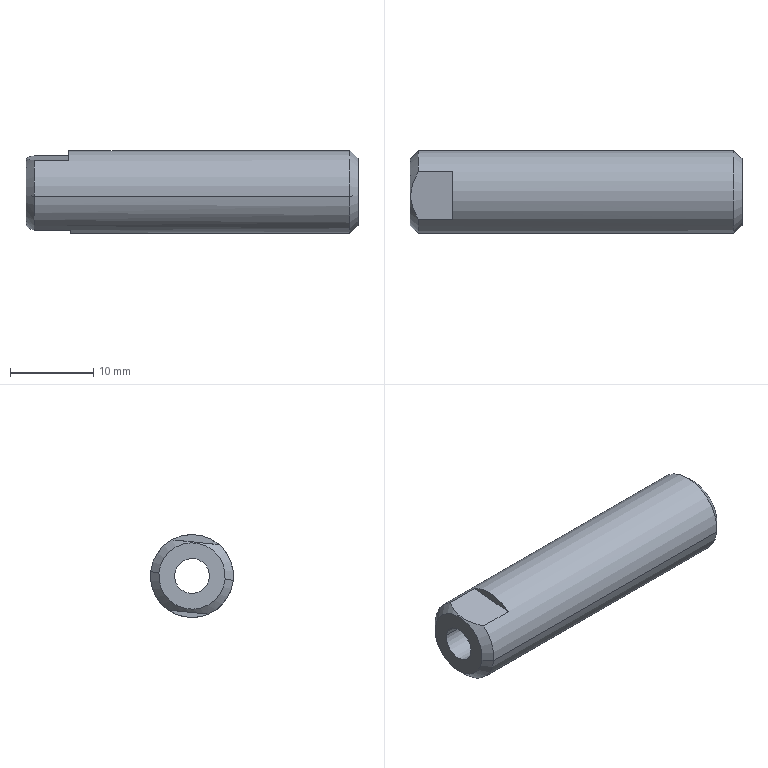Component | SolidWorks | CHEN123-AA-29-1 | 1 solid | 14 faces | box 40 x 10 x 10 mm | volume 2533 mm3 | plane 6 | cylinder 4 | cone 4 | commonest cylinder face diameters 4.2 x2 10 x2
build123d program:
from build123d import *

# Parameters (mm, degrees)
SKETCH1_R               = 5
BOSS_EXTRUDE1_DEPTH     = 40
CHAMFER1_SIZE           = 1
CUT_EXTRUDE1_DEPTH      = 41.62
CUT_EXTRUDE1_DEPTH_BACK = 41.62
SKETCH2_W               = 12.006
SKETCH2_H               = 4.106
SKETCH2_W_2             = 11.65
SKETCH2_H_2             = 2.222
M5_TAPPED_HOLE1_D       = 4.2


with BuildPart() as part:
    # Sketch1 → Boss-Extrude1 (new body)
    with BuildSketch(Plane.XY):
        Circle(SKETCH1_R)
    extrude(amount=BOSS_EXTRUDE1_DEPTH)

    # Chamfer1
    chamfer1_edges = [part.edges().sort_by_distance(p)[0] for p in [
        (-5, 0, 0),
        (-5, 0, 40),
    ]]
    chamfer(chamfer1_edges, length=CHAMFER1_SIZE)

    # Sketch2 → Cut-Extrude1 (cut, two sides: drawn at the far end of the back side and taken through both)
    with BuildSketch(Plane(origin=(0, 0, 0), x_dir=(0, 0, -1), z_dir=(1, 0, 0)).offset(-CUT_EXTRUDE1_DEPTH_BACK)):
        with Locations((-40.625, 6.426)):
            Rectangle(SKETCH2_W, SKETCH2_H)
        with Locations((-40.659, -5.201)):
            Rectangle(SKETCH2_W_2, SKETCH2_H_2)
    extrude(amount=CUT_EXTRUDE1_DEPTH + CUT_EXTRUDE1_DEPTH_BACK, mode=Mode.SUBTRACT)

    # M5 Tapped Hole1 (through all)
    with Locations(Plane.XY.offset(40)):
        with Locations((0, 0)):
            Hole(M5_TAPPED_HOLE1_D / 2)


solid = part.part

# Placed as in the assembly
solid = solid.moved(Location((20, -45.999, -230), (-167.254, -90, -83.091)))
STEP:
#1=COLOUR_RGB('',0.7922,0.8196,0.9333);
#2=FILL_AREA_STYLE_COLOUR('',#1);
#3=FILL_AREA_STYLE('',(#2));
#4=SURFACE_STYLE_FILL_AREA(#3);
#5=SURFACE_SIDE_STYLE('',(#4));
#6=SURFACE_STYLE_USAGE(.BOTH.,#5);
#7=PRESENTATION_STYLE_ASSIGNMENT((#6));
#8=CARTESIAN_POINT('',(0.7874,-1.893,-9.064));
#9=VERTEX_POINT('',#8);
#10=CARTESIAN_POINT('',(0.7874,-1.729,-9.047));
#11=VERTEX_POINT('',#10);
#12=CARTESIAN_POINT('',(0.7874,-1.811,-9.055));
#13=DIRECTION('',(-1.,0.,0.));
#14=DIRECTION('',(0.,0.9948,0.1017));
#15=AXIS2_PLACEMENT_3D('',#12,#13,#14);
#16=CIRCLE('',#15,0.08268);
#17=EDGE_CURVE('',#9,#11,#16,.T.);
#18=ORIENTED_EDGE('',*,*,#17,.F.);
#19=CARTESIAN_POINT('',(-0.7874,-1.893,-9.064));
#20=VERTEX_POINT('',#19);
#21=CARTESIAN_POINT('',(-0.7874,-1.893,-9.064));
#22=DIRECTION('',(-1.,0.,0.));
#23=VECTOR('',#22,39.37);
#24=LINE('',#21,#23);
#25=EDGE_CURVE('',#9,#20,#24,.T.);
#26=ORIENTED_EDGE('',*,*,#25,.T.);
#27=CARTESIAN_POINT('',(-0.7874,-1.729,-9.047));
#28=VERTEX_POINT('',#27);
#29=CARTESIAN_POINT('',(-0.7874,-1.811,-9.055));
#30=DIRECTION('',(-1.,0.,0.));
#31=DIRECTION('',(0.,0.9948,0.1017));
#32=AXIS2_PLACEMENT_3D('',#29,#30,#31);
#33=CIRCLE('',#32,0.08268);
#34=EDGE_CURVE('',#20,#28,#33,.T.);
#35=ORIENTED_EDGE('',*,*,#34,.T.);
#36=CARTESIAN_POINT('',(-0.7874,-1.729,-9.047));
#37=DIRECTION('',(-1.,0.,0.));
#38=VECTOR('',#37,39.37);
#39=LINE('',#36,#38);
#40=EDGE_CURVE('',#11,#28,#39,.T.);
#41=ORIENTED_EDGE('',*,*,#40,.F.);
#42=EDGE_LOOP('',(#18,#26,#35,#41));
#43=FACE_OUTER_BOUND('',#42,.T.);
#44=CARTESIAN_POINT('',(-0.7874,-1.811,-9.055));
#45=DIRECTION('',(-1.,0.,0.));
#46=DIRECTION('',(0.,0.9948,0.1017));
#47=AXIS2_PLACEMENT_3D('',#44,#45,#46);
#48=CYLINDRICAL_SURFACE('',#47,0.08268);
#49=ADVANCED_FACE('',(#43),#48,.F.);
#50=CARTESIAN_POINT('',(-0.7874,-1.654,-9.039));
#51=VERTEX_POINT('',#50);
#52=CARTESIAN_POINT('',(-0.7874,-1.968,-9.071));
#53=VERTEX_POINT('',#52);
#54=CARTESIAN_POINT('',(-0.7874,-1.811,-9.055));
#55=DIRECTION('',(-1.,0.,0.));
#56=DIRECTION('',(0.,0.9948,0.1017));
#57=AXIS2_PLACEMENT_3D('',#54,#55,#56);
#58=CIRCLE('',#57,0.1575);
#59=EDGE_CURVE('',#51,#53,#58,.T.);
#60=ORIENTED_EDGE('',*,*,#59,.F.);
#61=CARTESIAN_POINT('',(-0.7481,-1.615,-9.035));
#62=VERTEX_POINT('',#61);
#63=CARTESIAN_POINT('',(-0.7874,-1.654,-9.039));
#64=DIRECTION('',(0.7071,0.7034,0.07191));
#65=VECTOR('',#64,39.37);
#66=LINE('',#63,#65);
#67=EDGE_CURVE('',#51,#62,#66,.T.);
#68=ORIENTED_EDGE('',*,*,#67,.T.);
#69=CARTESIAN_POINT('',(-0.7481,-1.699,-9.217));
#70=VERTEX_POINT('',#69);
#71=CARTESIAN_POINT('',(-0.7481,-1.811,-9.055));
#72=DIRECTION('',(1.,0.,0.));
#73=DIRECTION('',(0.,0.9948,0.1017));
#74=AXIS2_PLACEMENT_3D('',#71,#72,#73);
#75=CIRCLE('',#74,0.1969);
#76=EDGE_CURVE('',#70,#62,#75,.T.);
#77=ORIENTED_EDGE('',*,*,#76,.F.);
#78=CARTESIAN_POINT('',(-0.7481,-1.888,-9.236));
#79=VERTEX_POINT('',#78);
#80=CARTESIAN_POINT('',(-0.7481,-1.888,-9.236));
#81=CARTESIAN_POINT('',(-0.7552,-1.874,-9.235));
#82=CARTESIAN_POINT('',(-0.7615,-1.858,-9.233));
#83=CARTESIAN_POINT('',(-0.7702,-1.826,-9.23));
#84=CARTESIAN_POINT('',(-0.7727,-1.81,-9.228));
#85=CARTESIAN_POINT('',(-0.7727,-1.777,-9.225));
#86=CARTESIAN_POINT('',(-0.7702,-1.761,-9.223));
#87=CARTESIAN_POINT('',(-0.7637,-1.737,-9.221));
#88=CARTESIAN_POINT('',(-0.761,-1.729,-9.22));
#89=CARTESIAN_POINT('',(-0.755,-1.713,-9.218));
#90=CARTESIAN_POINT('',(-0.7516,-1.706,-9.217));
#91=CARTESIAN_POINT('',(-0.7481,-1.699,-9.217));
#92=B_SPLINE_CURVE_WITH_KNOTS('',3,(#80,#81,#82,#83,#84,#85,#86,#87,#88,#89,#90,#91),.UNSPECIFIED.,.F.,.F.,(4,2,2,2,2,4),(0.003135,0.004387,0.005639,0.006891,0.007517,0.008143),.UNSPECIFIED.);
#93=EDGE_CURVE('',#79,#70,#92,.T.);
#94=ORIENTED_EDGE('',*,*,#93,.F.);
#95=CARTESIAN_POINT('',(-0.7481,-2.007,-9.075));
#96=VERTEX_POINT('',#95);
#97=CARTESIAN_POINT('',(-0.7481,-1.811,-9.055));
#98=DIRECTION('',(1.,0.,0.));
#99=DIRECTION('',(0.,0.9948,0.1017));
#100=AXIS2_PLACEMENT_3D('',#97,#98,#99);
#101=CIRCLE('',#100,0.1969);
#102=EDGE_CURVE('',#96,#79,#101,.T.);
#103=ORIENTED_EDGE('',*,*,#102,.F.);
#104=CARTESIAN_POINT('',(-0.7874,-1.968,-9.071));
#105=DIRECTION('',(0.7071,-0.7034,-0.07191));
#106=VECTOR('',#105,39.37);
#107=LINE('',#104,#106);
#108=EDGE_CURVE('',#53,#96,#107,.T.);
#109=ORIENTED_EDGE('',*,*,#108,.F.);
#110=EDGE_LOOP('',(#60,#68,#77,#94,#103,#109));
#111=FACE_OUTER_BOUND('',#110,.T.);
#112=CARTESIAN_POINT('',(-0.7874,-1.811,-9.055));
#113=DIRECTION('',(1.,0.,0.));
#114=DIRECTION('',(0.,-0.9948,-0.1017));
#115=AXIS2_PLACEMENT_3D('',#112,#113,#114);
#116=CONICAL_SURFACE('',#115,0.1575,0.7854);
#117=ADVANCED_FACE('',(#111),#116,.T.);
#118=CARTESIAN_POINT('',(0.7874,-1.968,-9.071));
#119=VERTEX_POINT('',#118);
#120=CARTESIAN_POINT('',(0.7874,-1.654,-9.039));
#121=VERTEX_POINT('',#120);
#122=CARTESIAN_POINT('',(0.7874,-1.811,-9.055));
#123=DIRECTION('',(1.,0.,0.));
#124=DIRECTION('',(0.,0.9948,0.1017));
#125=AXIS2_PLACEMENT_3D('',#122,#123,#124);
#126=CIRCLE('',#125,0.1575);
#127=EDGE_CURVE('',#119,#121,#126,.T.);
#128=ORIENTED_EDGE('',*,*,#127,.F.);
#129=CARTESIAN_POINT('',(0.748,-2.007,-9.075));
#130=VERTEX_POINT('',#129);
#131=CARTESIAN_POINT('',(0.748,-2.007,-9.075));
#132=DIRECTION('',(-0.7071,-0.7034,-0.07191));
#133=VECTOR('',#132,39.37);
#134=LINE('',#131,#133);
#135=EDGE_CURVE('',#119,#130,#134,.T.);
#136=ORIENTED_EDGE('',*,*,#135,.T.);
#137=CARTESIAN_POINT('',(0.748,-1.615,-9.035));
#138=VERTEX_POINT('',#137);
#139=CARTESIAN_POINT('',(0.748,-1.811,-9.055));
#140=DIRECTION('',(-1.,0.,0.));
#141=DIRECTION('',(0.,0.9948,0.1017));
#142=AXIS2_PLACEMENT_3D('',#139,#140,#141);
#143=CIRCLE('',#142,0.1969);
#144=EDGE_CURVE('',#138,#130,#143,.T.);
#145=ORIENTED_EDGE('',*,*,#144,.F.);
#146=CARTESIAN_POINT('',(0.748,-1.615,-9.035));
#147=DIRECTION('',(-0.7071,0.7034,0.07191));
#148=VECTOR('',#147,39.37);
#149=LINE('',#146,#148);
#150=EDGE_CURVE('',#121,#138,#149,.T.);
#151=ORIENTED_EDGE('',*,*,#150,.F.);
#152=EDGE_LOOP('',(#128,#136,#145,#151));
#153=FACE_OUTER_BOUND('',#152,.T.);
#154=CARTESIAN_POINT('',(0.748,-1.811,-9.055));
#155=DIRECTION('',(-1.,0.,0.));
#156=DIRECTION('',(0.,0.9948,0.1017));
#157=AXIS2_PLACEMENT_3D('',#154,#155,#156);
#158=CONICAL_SURFACE('',#157,0.1969,0.7854);
#159=ADVANCED_FACE('',(#153),#158,.T.);
#160=ORIENTED_EDGE('',*,*,#76,.T.);
#161=CARTESIAN_POINT('',(-0.7874,-1.615,-9.035));
#162=DIRECTION('',(1.,0.,0.));
#163=VECTOR('',#162,39.37);
#164=LINE('',#161,#163);
#165=EDGE_CURVE('',#62,#138,#164,.T.);
#166=ORIENTED_EDGE('',*,*,#165,.T.);
#167=ORIENTED_EDGE('',*,*,#144,.T.);
#168=CARTESIAN_POINT('',(-0.7874,-2.007,-9.075));
#169=DIRECTION('',(1.,0.,0.));
#170=VECTOR('',#169,39.37);
#171=LINE('',#168,#170);
#172=EDGE_CURVE('',#96,#130,#171,.T.);
#173=ORIENTED_EDGE('',*,*,#172,.F.);
#174=ORIENTED_EDGE('',*,*,#102,.T.);
#175=CARTESIAN_POINT('',(-0.5757,-1.888,-9.236));
#176=VERTEX_POINT('',#175);
#177=CARTESIAN_POINT('',(-0.7874,-1.888,-9.236));
#178=DIRECTION('',(1.,0.,0.));
#179=VECTOR('',#178,39.37);
#180=LINE('',#177,#179);
#181=EDGE_CURVE('',#79,#176,#180,.T.);
#182=ORIENTED_EDGE('',*,*,#181,.T.);
#183=CARTESIAN_POINT('',(-0.5757,-1.699,-9.217));
#184=VERTEX_POINT('',#183);
#185=CARTESIAN_POINT('',(-0.5757,-1.811,-9.055));
#186=DIRECTION('',(1.,0.,0.));
#187=DIRECTION('',(0.,-0.9948,-0.1017));
#188=AXIS2_PLACEMENT_3D('',#185,#186,#187);
#189=CIRCLE('',#188,0.1969);
#190=EDGE_CURVE('',#176,#184,#189,.T.);
#191=ORIENTED_EDGE('',*,*,#190,.T.);
#192=CARTESIAN_POINT('',(-0.7874,-1.699,-9.217));
#193=DIRECTION('',(-1.,0.,0.));
#194=VECTOR('',#193,39.37);
#195=LINE('',#192,#194);
#196=EDGE_CURVE('',#184,#70,#195,.T.);
#197=ORIENTED_EDGE('',*,*,#196,.T.);
#198=EDGE_LOOP('',(#160,#166,#167,#173,#174,#182,#191,#197));
#199=FACE_OUTER_BOUND('',#198,.T.);
#200=CARTESIAN_POINT('',(-0.7874,-1.811,-9.055));
#201=DIRECTION('',(1.,0.,0.));
#202=DIRECTION('',(0.,-0.9948,-0.1017));
#203=AXIS2_PLACEMENT_3D('',#200,#201,#202);
#204=CYLINDRICAL_SURFACE('',#203,0.1969);
#205=ADVANCED_FACE('',(#199),#204,.T.);
#206=ORIENTED_EDGE('',*,*,#165,.F.);
#207=CARTESIAN_POINT('',(-0.7481,-1.715,-8.883));
#208=VERTEX_POINT('',#207);
#209=CARTESIAN_POINT('',(-0.7481,-1.811,-9.055));
#210=DIRECTION('',(1.,0.,0.));
#211=DIRECTION('',(0.,0.9948,0.1017));
#212=AXIS2_PLACEMENT_3D('',#209,#210,#211);
#213=CIRCLE('',#212,0.1969);
#214=EDGE_CURVE('',#62,#208,#213,.T.);
#215=ORIENTED_EDGE('',*,*,#214,.T.);
#216=CARTESIAN_POINT('',(-0.584,-1.715,-8.883));
#217=VERTEX_POINT('',#216);
#218=CARTESIAN_POINT('',(-0.7874,-1.715,-8.883));
#219=DIRECTION('',(1.,0.,0.));
#220=VECTOR('',#219,39.37);
#221=LINE('',#218,#220);
#222=EDGE_CURVE('',#208,#217,#221,.T.);
#223=ORIENTED_EDGE('',*,*,#222,.T.);
#224=CARTESIAN_POINT('',(-0.584,-1.94,-8.906));
#225=VERTEX_POINT('',#224);
#226=CARTESIAN_POINT('',(-0.584,-1.811,-9.055));
#227=DIRECTION('',(1.,0.,0.));
#228=DIRECTION('',(0.,-0.9948,-0.1017));
#229=AXIS2_PLACEMENT_3D('',#226,#227,#228);
#230=CIRCLE('',#229,0.1969);
#231=EDGE_CURVE('',#217,#225,#230,.T.);
#232=ORIENTED_EDGE('',*,*,#231,.T.);
#233=CARTESIAN_POINT('',(-0.7481,-1.94,-8.906));
#234=VERTEX_POINT('',#233);
#235=CARTESIAN_POINT('',(-0.7874,-1.94,-8.906));
#236=DIRECTION('',(-1.,0.,0.));
#237=VECTOR('',#236,39.37);
#238=LINE('',#235,#237);
#239=EDGE_CURVE('',#225,#234,#238,.T.);
#240=ORIENTED_EDGE('',*,*,#239,.T.);
#241=CARTESIAN_POINT('',(-0.7481,-1.811,-9.055));
#242=DIRECTION('',(1.,0.,0.));
#243=DIRECTION('',(0.,0.9948,0.1017));
#244=AXIS2_PLACEMENT_3D('',#241,#242,#243);
#245=CIRCLE('',#244,0.1969);
#246=EDGE_CURVE('',#234,#96,#245,.T.);
#247=ORIENTED_EDGE('',*,*,#246,.T.);
#248=ORIENTED_EDGE('',*,*,#172,.T.);
#249=CARTESIAN_POINT('',(0.748,-1.811,-9.055));
#250=DIRECTION('',(-1.,0.,0.));
#251=DIRECTION('',(0.,0.9948,0.1017));
#252=AXIS2_PLACEMENT_3D('',#249,#250,#251);
#253=CIRCLE('',#252,0.1969);
#254=EDGE_CURVE('',#130,#138,#253,.T.);
#255=ORIENTED_EDGE('',*,*,#254,.T.);
#256=EDGE_LOOP('',(#206,#215,#223,#232,#240,#247,#248,#255));
#257=FACE_OUTER_BOUND('',#256,.T.);
#258=CARTESIAN_POINT('',(-0.7874,-1.811,-9.055));
#259=DIRECTION('',(1.,0.,0.));
#260=DIRECTION('',(0.,-0.9948,-0.1017));
#261=AXIS2_PLACEMENT_3D('',#258,#259,#260);
#262=CYLINDRICAL_SURFACE('',#261,0.1969);
#263=ADVANCED_FACE('',(#257),#262,.T.);
#264=CARTESIAN_POINT('',(-0.7874,-1.811,-9.055));
#265=DIRECTION('',(-1.,0.,0.));
#266=DIRECTION('',(0.,0.9948,0.1017));
#267=AXIS2_PLACEMENT_3D('',#264,#265,#266);
#268=CIRCLE('',#267,0.08268);
#269=EDGE_CURVE('',#28,#20,#268,.T.);
#270=ORIENTED_EDGE('',*,*,#269,.F.);
#271=ORIENTED_EDGE('',*,*,#34,.F.);
#272=EDGE_LOOP('',(#270,#271));
#273=FACE_BOUND('',#272,.T.);
#274=CARTESIAN_POINT('',(-0.7874,-1.811,-9.055));
#275=DIRECTION('',(-1.,0.,0.));
#276=DIRECTION('',(0.,0.9948,0.1017));
#277=AXIS2_PLACEMENT_3D('',#274,#275,#276);
#278=CIRCLE('',#277,0.1575);
#279=EDGE_CURVE('',#53,#51,#278,.T.);
#280=ORIENTED_EDGE('',*,*,#279,.T.);
#281=ORIENTED_EDGE('',*,*,#59,.T.);
#282=EDGE_LOOP('',(#280,#281));
#283=FACE_OUTER_BOUND('',#282,.T.);
#284=CARTESIAN_POINT('',(-0.7874,-1.811,-9.055));
#285=DIRECTION('',(-1.,0.,0.));
#286=DIRECTION('',(0.,0.9948,0.1017));
#287=AXIS2_PLACEMENT_3D('',#284,#285,#286);
#288=PLANE('',#287);
#289=ADVANCED_FACE('',(#273,#283),#288,.T.);
#290=CARTESIAN_POINT('',(0.7874,-1.811,-9.055));
#291=DIRECTION('',(-1.,0.,0.));
#292=DIRECTION('',(0.,0.9948,0.1017));
#293=AXIS2_PLACEMENT_3D('',#290,#291,#292);
#294=CIRCLE('',#293,0.08268);
#295=EDGE_CURVE('',#11,#9,#294,.T.);
#296=ORIENTED_EDGE('',*,*,#295,.T.);
#297=ORIENTED_EDGE('',*,*,#17,.T.);
#298=EDGE_LOOP('',(#296,#297));
#299=FACE_BOUND('',#298,.T.);
#300=CARTESIAN_POINT('',(0.7874,-1.811,-9.055));
#301=DIRECTION('',(1.,0.,0.));
#302=DIRECTION('',(0.,0.9948,0.1017));
#303=AXIS2_PLACEMENT_3D('',#300,#301,#302);
#304=CIRCLE('',#303,0.1575);
#305=EDGE_CURVE('',#121,#119,#304,.T.);
#306=ORIENTED_EDGE('',*,*,#305,.T.);
#307=ORIENTED_EDGE('',*,*,#127,.T.);
#308=EDGE_LOOP('',(#306,#307));
#309=FACE_OUTER_BOUND('',#308,.T.);
#310=CARTESIAN_POINT('',(0.7874,-1.811,-9.055));
#311=DIRECTION('',(-1.,0.,0.));
#312=DIRECTION('',(0.,0.9948,0.1017));
#313=AXIS2_PLACEMENT_3D('',#310,#311,#312);
#314=PLANE('',#313);
#315=ADVANCED_FACE('',(#299,#309),#314,.F.);
#316=ORIENTED_EDGE('',*,*,#135,.F.);
#317=ORIENTED_EDGE('',*,*,#305,.F.);
#318=ORIENTED_EDGE('',*,*,#150,.T.);
#319=ORIENTED_EDGE('',*,*,#254,.F.);
#320=EDGE_LOOP('',(#316,#317,#318,#319));
#321=FACE_OUTER_BOUND('',#320,.T.);
#322=CARTESIAN_POINT('',(0.748,-1.811,-9.055));
#323=DIRECTION('',(-1.,0.,0.));
#324=DIRECTION('',(0.,0.9948,0.1017));
#325=AXIS2_PLACEMENT_3D('',#322,#323,#324);
#326=CONICAL_SURFACE('',#325,0.1969,0.7854);
#327=ADVANCED_FACE('',(#321),#326,.T.);
#328=ORIENTED_EDGE('',*,*,#67,.F.);
#329=ORIENTED_EDGE('',*,*,#279,.F.);
#330=ORIENTED_EDGE('',*,*,#108,.T.);
#331=ORIENTED_EDGE('',*,*,#246,.F.);
#332=CARTESIAN_POINT('',(-0.7481,-1.715,-8.883));
#333=CARTESIAN_POINT('',(-0.753,-1.723,-8.884));
#334=CARTESIAN_POINT('',(-0.7577,-1.732,-8.885));
#335=CARTESIAN_POINT('',(-0.7662,-1.75,-8.887));
#336=CARTESIAN_POINT('',(-0.7701,-1.759,-8.888));
#337=CARTESIAN_POINT('',(-0.7767,-1.778,-8.89));
#338=CARTESIAN_POINT('',(-0.7793,-1.788,-8.891));
#339=CARTESIAN_POINT('',(-0.7829,-1.807,-8.893));
#340=CARTESIAN_POINT('',(-0.7839,-1.817,-8.894));
#341=CARTESIAN_POINT('',(-0.7839,-1.837,-8.896));
#342=CARTESIAN_POINT('',(-0.7829,-1.847,-8.897));
#343=CARTESIAN_POINT('',(-0.7793,-1.867,-8.899));
#344=CARTESIAN_POINT('',(-0.7767,-1.877,-8.9));
#345=CARTESIAN_POINT('',(-0.7669,-1.905,-8.903));
#346=CARTESIAN_POINT('',(-0.758,-1.923,-8.905));
#347=CARTESIAN_POINT('',(-0.7481,-1.94,-8.906));
#348=B_SPLINE_CURVE_WITH_KNOTS('',3,(#332,#333,#334,#335,#336,#337,#338,#339,#340,#341,#342,#343,#344,#345,#346,#347),.UNSPECIFIED.,.F.,.F.,(4,2,2,2,2,2,2,4),(0.002509,0.003265,0.004021,0.004778,0.005534,0.006291,0.007047,0.00856),.UNSPECIFIED.);
#349=EDGE_CURVE('',#208,#234,#348,.T.);
#350=ORIENTED_EDGE('',*,*,#349,.F.);
#351=ORIENTED_EDGE('',*,*,#214,.F.);
#352=EDGE_LOOP('',(#328,#329,#330,#331,#350,#351));
#353=FACE_OUTER_BOUND('',#352,.T.);
#354=CARTESIAN_POINT('',(-0.7874,-1.811,-9.055));
#355=DIRECTION('',(1.,0.,0.));
#356=DIRECTION('',(0.,-0.9948,-0.1017));
#357=AXIS2_PLACEMENT_3D('',#354,#355,#356);
#358=CONICAL_SURFACE('',#357,0.1575,0.7854);
#359=ADVANCED_FACE('',(#353),#358,.T.);
#360=CARTESIAN_POINT('',(-0.584,-2.023,-8.915));
#361=DIRECTION('',(0.,0.9948,0.1017));
#362=VECTOR('',#361,39.37);
#363=LINE('',#360,#362);
#364=EDGE_CURVE('',#225,#217,#363,.T.);
#365=ORIENTED_EDGE('',*,*,#364,.F.);
#366=ORIENTED_EDGE('',*,*,#231,.F.);
#367=EDGE_LOOP('',(#365,#366));
#368=FACE_OUTER_BOUND('',#367,.T.);
#369=CARTESIAN_POINT('',(-0.584,-2.023,-8.915));
#370=DIRECTION('',(1.,0.,0.));
#371=DIRECTION('',(0.,-0.9948,-0.1017));
#372=AXIS2_PLACEMENT_3D('',#369,#370,#371);
#373=PLANE('',#372);
#374=ADVANCED_FACE('',(#368),#373,.F.);
#375=ORIENTED_EDGE('',*,*,#349,.T.);
#376=ORIENTED_EDGE('',*,*,#239,.F.);
#377=ORIENTED_EDGE('',*,*,#364,.T.);
#378=ORIENTED_EDGE('',*,*,#222,.F.);
#379=EDGE_LOOP('',(#375,#376,#377,#378));
#380=FACE_OUTER_BOUND('',#379,.T.);
#381=CARTESIAN_POINT('',(-1.043,-2.023,-8.915));
#382=DIRECTION('',(0.,0.1017,-0.9948));
#383=DIRECTION('',(-1.,0.,0.));
#384=AXIS2_PLACEMENT_3D('',#381,#382,#383);
#385=PLANE('',#384);
#386=ADVANCED_FACE('',(#380),#385,.F.);
#387=CARTESIAN_POINT('',(-0.5757,-1.989,-9.246));
#388=DIRECTION('',(0.,0.9948,0.1017));
#389=VECTOR('',#388,39.37);
#390=LINE('',#387,#389);
#391=EDGE_CURVE('',#176,#184,#390,.T.);
#392=ORIENTED_EDGE('',*,*,#391,.T.);
#393=ORIENTED_EDGE('',*,*,#190,.F.);
#394=EDGE_LOOP('',(#392,#393));
#395=FACE_OUTER_BOUND('',#394,.T.);
#396=CARTESIAN_POINT('',(-0.5757,-1.973,-9.407));
#397=DIRECTION('',(1.,0.,0.));
#398=DIRECTION('',(0.,-0.9948,-0.1017));
#399=AXIS2_PLACEMENT_3D('',#396,#397,#398);
#400=PLANE('',#399);
#401=ADVANCED_FACE('',(#395),#400,.F.);
#402=ORIENTED_EDGE('',*,*,#93,.T.);
#403=ORIENTED_EDGE('',*,*,#196,.F.);
#404=ORIENTED_EDGE('',*,*,#391,.F.);
#405=ORIENTED_EDGE('',*,*,#181,.F.);
#406=EDGE_LOOP('',(#402,#403,#404,#405));
#407=FACE_OUTER_BOUND('',#406,.T.);
#408=CARTESIAN_POINT('',(-1.048,-1.989,-9.246));
#409=DIRECTION('',(0.,-0.1017,0.9948));
#410=DIRECTION('',(1.,0.,0.));
#411=AXIS2_PLACEMENT_3D('',#408,#409,#410);
#412=PLANE('',#411);
#413=ADVANCED_FACE('',(#407),#412,.F.);
#414=ORIENTED_EDGE('',*,*,#25,.F.);
#415=ORIENTED_EDGE('',*,*,#295,.F.);
#416=ORIENTED_EDGE('',*,*,#40,.T.);
#417=ORIENTED_EDGE('',*,*,#269,.T.);
#418=EDGE_LOOP('',(#414,#415,#416,#417));
#419=FACE_OUTER_BOUND('',#418,.T.);
#420=CARTESIAN_POINT('',(-0.7874,-1.811,-9.055));
#421=DIRECTION('',(-1.,0.,0.));
#422=DIRECTION('',(0.,0.9948,0.1017));
#423=AXIS2_PLACEMENT_3D('',#420,#421,#422);
#424=CYLINDRICAL_SURFACE('',#423,0.08268);
#425=ADVANCED_FACE('',(#419),#424,.F.);
#426=CLOSED_SHELL('',(#49,#117,#159,#205,#263,#289,#315,#327,#359,#374,#386,#401,#413,#425));
#427=MANIFOLD_SOLID_BREP('',#426);
#428=STYLED_ITEM('',(#7),#427);
#429=PRESENTATION_LAYER_ASSIGNMENT('','',(#428));
#430=CARTESIAN_POINT('',(0.,0.,0.));
#431=DIRECTION('',(0.,0.,1.));
#432=DIRECTION('',(1.,0.,0.));
#433=AXIS2_PLACEMENT_3D('',#430,#431,#432);
#434=(LENGTH_UNIT()NAMED_UNIT(*)SI_UNIT($,.METRE.));
#435=LENGTH_MEASURE_WITH_UNIT(LENGTH_MEASURE(0.0254),#434);
#436=DIMENSIONAL_EXPONENTS(1.,0.,0.,0.,0.,0.,0.);
#437=(CONVERSION_BASED_UNIT('',#435)LENGTH_UNIT()NAMED_UNIT(#436));
#438=UNCERTAINTY_MEASURE_WITH_UNIT(LENGTH_MEASURE(0.00001),#437,'','');
#439=(NAMED_UNIT(*)PLANE_ANGLE_UNIT()SI_UNIT($,.RADIAN.));
#440=(NAMED_UNIT(*)SI_UNIT($,.STERADIAN.)SOLID_ANGLE_UNIT());
#441=(GEOMETRIC_REPRESENTATION_CONTEXT(3)GLOBAL_UNCERTAINTY_ASSIGNED_CONTEXT((#438))GLOBAL_UNIT_ASSIGNED_CONTEXT((#437,#439,#440))REPRESENTATION_CONTEXT('',''));
#442=ADVANCED_BREP_SHAPE_REPRESENTATION('',(#427,#433),#441);
#443=(LENGTH_UNIT()NAMED_UNIT(*)SI_UNIT($,.METRE.));
#444=LENGTH_MEASURE_WITH_UNIT(LENGTH_MEASURE(0.0254),#443);
#445=DIMENSIONAL_EXPONENTS(1.,0.,0.,0.,0.,0.,0.);
#446=(CONVERSION_BASED_UNIT('',#444)LENGTH_UNIT()NAMED_UNIT(#445));
#447=UNCERTAINTY_MEASURE_WITH_UNIT(LENGTH_MEASURE(0.00001),#446,'','');
#448=(NAMED_UNIT(*)PLANE_ANGLE_UNIT()SI_UNIT($,.RADIAN.));
#449=(NAMED_UNIT(*)SI_UNIT($,.STERADIAN.)SOLID_ANGLE_UNIT());
#450=(GEOMETRIC_REPRESENTATION_CONTEXT(3)GLOBAL_UNCERTAINTY_ASSIGNED_CONTEXT((#447))GLOBAL_UNIT_ASSIGNED_CONTEXT((#446,#448,#449))REPRESENTATION_CONTEXT('',''));
#451=MECHANICAL_DESIGN_GEOMETRIC_PRESENTATION_REPRESENTATION('',(#428),#450);